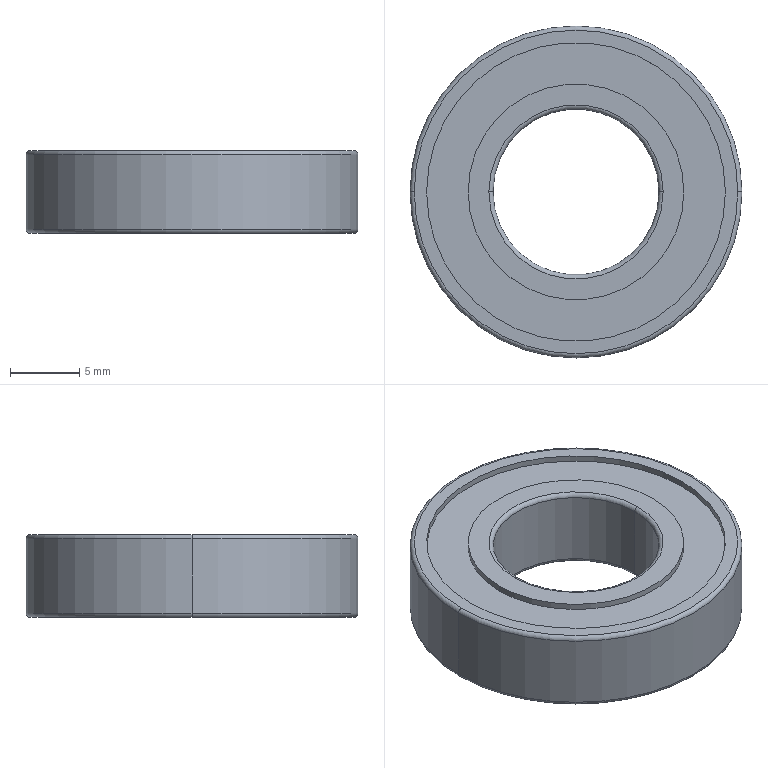Component | SolidWorks | TensioningWheel-2-1_B6901ZZ-2-2 | 1 solid | 26 faces | box 24 x 24 x 6 mm | volume 1874 mm3 | cylinder 12 | torus 8 | plane 6 | commonest cylinder face diameters 21.6 x4 15.6 x4 24 x2 12 x2
build123d program:
from build123d import *


with BuildPart() as part:
    # Sketch1 → Revolve1 (revolve)
    with BuildSketch(Plane.XY, mode=Mode.PRIVATE) as revolve1_sk:
        with BuildLine():
            Line((0, 11.7), (0, 10.8))
            Line((0, 10.8), (0.45, 10.8))
            Line((0.45, 10.8), (0.45, 7.8))
            Line((0.45, 7.8), (0, 7.8))
            Line((0, 7.8), (0, 6.3))
            ThreePointArc((0, 6.3), (0.08787, 6.088), (0.3, 6))
            Line((0.3, 6), (5.7, 6))
            ThreePointArc((5.7, 6), (5.912, 6.088), (6, 6.3))
            Line((6, 6.3), (6, 7.8))
            Line((6, 7.8), (5.55, 7.8))
            Line((5.55, 7.8), (5.55, 10.8))
            Line((5.55, 10.8), (6, 10.8))
            Line((6, 10.8), (6, 11.7))
            ThreePointArc((6, 11.7), (5.912, 11.912), (5.7, 12))
            Line((5.7, 12), (0.3, 12))
            ThreePointArc((0.3, 12), (0.08787, 11.912), (0, 11.7))
        make_face()
    revolve(revolve1_sk.sketch.rotate(Axis((6, 0, 0), (-1, 0, 0)), 270), axis=Axis((6, 0, 0), (-1, 0, 0)))


solid = part.part

# Placed as in the assembly
solid = solid.moved(Location((538.036, -118.615, -116), (0, 90, 0)))
STEP:
#1=COLOUR_RGB('',0.7922,0.8196,0.9333);
#2=FILL_AREA_STYLE_COLOUR('',#1);
#3=FILL_AREA_STYLE('',(#2));
#4=SURFACE_STYLE_FILL_AREA(#3);
#5=SURFACE_SIDE_STYLE('',(#4));
#6=SURFACE_STYLE_USAGE(.BOTH.,#5);
#7=PRESENTATION_STYLE_ASSIGNMENT((#6));
#8=CARTESIAN_POINT('',(20.71,-4.67,-4.579));
#9=VERTEX_POINT('',#8);
#10=CARTESIAN_POINT('',(21.655,-4.67,-4.579));
#11=VERTEX_POINT('',#10);
#12=CARTESIAN_POINT('',(21.183,-4.67,-4.579));
#13=DIRECTION('',(0.,0.,-1.));
#14=DIRECTION('',(-1.,0.,0.));
#15=AXIS2_PLACEMENT_3D('',#12,#13,#14);
#16=CIRCLE('',#15,0.4724);
#17=EDGE_CURVE('',#9,#11,#16,.T.);
#18=ORIENTED_EDGE('',*,*,#17,.T.);
#19=CARTESIAN_POINT('',(21.655,-4.67,-4.791));
#20=VERTEX_POINT('',#19);
#21=CARTESIAN_POINT('',(21.655,-4.67,-4.567));
#22=DIRECTION('',(0.,0.,-1.));
#23=VECTOR('',#22,39.37);
#24=LINE('',#21,#23);
#25=EDGE_CURVE('',#11,#20,#24,.T.);
#26=ORIENTED_EDGE('',*,*,#25,.T.);
#27=CARTESIAN_POINT('',(20.71,-4.67,-4.791));
#28=VERTEX_POINT('',#27);
#29=CARTESIAN_POINT('',(21.183,-4.67,-4.791));
#30=DIRECTION('',(0.,0.,-1.));
#31=DIRECTION('',(-1.,0.,0.));
#32=AXIS2_PLACEMENT_3D('',#29,#30,#31);
#33=CIRCLE('',#32,0.4724);
#34=EDGE_CURVE('',#28,#20,#33,.T.);
#35=ORIENTED_EDGE('',*,*,#34,.F.);
#36=CARTESIAN_POINT('',(20.71,-4.67,-4.567));
#37=DIRECTION('',(0.,0.,-1.));
#38=VECTOR('',#37,39.37);
#39=LINE('',#36,#38);
#40=EDGE_CURVE('',#9,#28,#39,.T.);
#41=ORIENTED_EDGE('',*,*,#40,.F.);
#42=EDGE_LOOP('',(#18,#26,#35,#41));
#43=FACE_OUTER_BOUND('',#42,.T.);
#44=CARTESIAN_POINT('',(21.183,-4.67,-4.567));
#45=DIRECTION('',(0.,0.,-1.));
#46=DIRECTION('',(-1.,0.,0.));
#47=AXIS2_PLACEMENT_3D('',#44,#45,#46);
#48=CYLINDRICAL_SURFACE('',#47,0.4724);
#49=ADVANCED_FACE('',(#43),#48,.T.);
#50=CARTESIAN_POINT('',(20.722,-4.67,-4.567));
#51=VERTEX_POINT('',#50);
#52=CARTESIAN_POINT('',(21.643,-4.67,-4.567));
#53=VERTEX_POINT('',#52);
#54=CARTESIAN_POINT('',(21.183,-4.67,-4.567));
#55=DIRECTION('',(0.,0.,-1.));
#56=DIRECTION('',(-1.,0.,0.));
#57=AXIS2_PLACEMENT_3D('',#54,#55,#56);
#58=CIRCLE('',#57,0.4606);
#59=EDGE_CURVE('',#51,#53,#58,.T.);
#60=ORIENTED_EDGE('',*,*,#59,.T.);
#61=CARTESIAN_POINT('',(21.643,-4.67,-4.579));
#62=DIRECTION('',(-0.,1.,0.));
#63=DIRECTION('',(-1.,0.,0.));
#64=AXIS2_PLACEMENT_3D('',#61,#62,#63);
#65=CIRCLE('',#64,0.01181);
#66=EDGE_CURVE('',#53,#11,#65,.T.);
#67=ORIENTED_EDGE('',*,*,#66,.T.);
#68=ORIENTED_EDGE('',*,*,#17,.F.);
#69=CARTESIAN_POINT('',(20.722,-4.67,-4.579));
#70=DIRECTION('',(-0.,-1.,-0.));
#71=DIRECTION('',(0.,0.,-1.));
#72=AXIS2_PLACEMENT_3D('',#69,#70,#71);
#73=CIRCLE('',#72,0.01181);
#74=EDGE_CURVE('',#51,#9,#73,.T.);
#75=ORIENTED_EDGE('',*,*,#74,.F.);
#76=EDGE_LOOP('',(#60,#67,#68,#75));
#77=FACE_OUTER_BOUND('',#76,.T.);
#78=CARTESIAN_POINT('',(21.183,-4.67,-4.579));
#79=DIRECTION('',(0.,0.,-1.));
#80=DIRECTION('',(-1.,0.,-0.));
#81=AXIS2_PLACEMENT_3D('',#78,#79,#80);
#82=TOROIDAL_SURFACE('',#81,0.4606,0.01181);
#83=ADVANCED_FACE('',(#77),#82,.T.);
#84=CARTESIAN_POINT('',(21.608,-4.67,-4.567));
#85=VERTEX_POINT('',#84);
#86=CARTESIAN_POINT('',(20.757,-4.67,-4.567));
#87=VERTEX_POINT('',#86);
#88=CARTESIAN_POINT('',(21.183,-4.67,-4.567));
#89=DIRECTION('',(0.,0.,-1.));
#90=DIRECTION('',(-1.,0.,0.));
#91=AXIS2_PLACEMENT_3D('',#88,#89,#90);
#92=CIRCLE('',#91,0.4252);
#93=EDGE_CURVE('',#85,#87,#92,.T.);
#94=ORIENTED_EDGE('',*,*,#93,.F.);
#95=CARTESIAN_POINT('',(21.608,-4.67,-4.585));
#96=VERTEX_POINT('',#95);
#97=CARTESIAN_POINT('',(21.608,-4.67,-4.567));
#98=DIRECTION('',(0.,0.,-1.));
#99=VECTOR('',#98,39.37);
#100=LINE('',#97,#99);
#101=EDGE_CURVE('',#85,#96,#100,.T.);
#102=ORIENTED_EDGE('',*,*,#101,.T.);
#103=CARTESIAN_POINT('',(20.757,-4.67,-4.585));
#104=VERTEX_POINT('',#103);
#105=CARTESIAN_POINT('',(21.183,-4.67,-4.585));
#106=DIRECTION('',(0.,0.,-1.));
#107=DIRECTION('',(-1.,0.,0.));
#108=AXIS2_PLACEMENT_3D('',#105,#106,#107);
#109=CIRCLE('',#108,0.4252);
#110=EDGE_CURVE('',#96,#104,#109,.T.);
#111=ORIENTED_EDGE('',*,*,#110,.T.);
#112=CARTESIAN_POINT('',(20.757,-4.67,-4.567));
#113=DIRECTION('',(0.,0.,-1.));
#114=VECTOR('',#113,39.37);
#115=LINE('',#112,#114);
#116=EDGE_CURVE('',#87,#104,#115,.T.);
#117=ORIENTED_EDGE('',*,*,#116,.F.);
#118=EDGE_LOOP('',(#94,#102,#111,#117));
#119=FACE_OUTER_BOUND('',#118,.T.);
#120=CARTESIAN_POINT('',(21.183,-4.67,-4.567));
#121=DIRECTION('',(0.,0.,-1.));
#122=DIRECTION('',(-1.,0.,0.));
#123=AXIS2_PLACEMENT_3D('',#120,#121,#122);
#124=CYLINDRICAL_SURFACE('',#123,0.4252);
#125=ADVANCED_FACE('',(#119),#124,.F.);
#126=CARTESIAN_POINT('',(20.875,-4.67,-4.567));
#127=VERTEX_POINT('',#126);
#128=CARTESIAN_POINT('',(21.49,-4.67,-4.567));
#129=VERTEX_POINT('',#128);
#130=CARTESIAN_POINT('',(21.183,-4.67,-4.567));
#131=DIRECTION('',(0.,0.,-1.));
#132=DIRECTION('',(-1.,0.,0.));
#133=AXIS2_PLACEMENT_3D('',#130,#131,#132);
#134=CIRCLE('',#133,0.3071);
#135=EDGE_CURVE('',#127,#129,#134,.T.);
#136=ORIENTED_EDGE('',*,*,#135,.T.);
#137=CARTESIAN_POINT('',(21.49,-4.67,-4.585));
#138=VERTEX_POINT('',#137);
#139=CARTESIAN_POINT('',(21.49,-4.67,-4.567));
#140=DIRECTION('',(0.,0.,-1.));
#141=VECTOR('',#140,39.37);
#142=LINE('',#139,#141);
#143=EDGE_CURVE('',#129,#138,#142,.T.);
#144=ORIENTED_EDGE('',*,*,#143,.T.);
#145=CARTESIAN_POINT('',(20.875,-4.67,-4.585));
#146=VERTEX_POINT('',#145);
#147=CARTESIAN_POINT('',(21.183,-4.67,-4.585));
#148=DIRECTION('',(0.,0.,-1.));
#149=DIRECTION('',(-1.,0.,0.));
#150=AXIS2_PLACEMENT_3D('',#147,#148,#149);
#151=CIRCLE('',#150,0.3071);
#152=EDGE_CURVE('',#146,#138,#151,.T.);
#153=ORIENTED_EDGE('',*,*,#152,.F.);
#154=CARTESIAN_POINT('',(20.875,-4.67,-4.567));
#155=DIRECTION('',(0.,0.,-1.));
#156=VECTOR('',#155,39.37);
#157=LINE('',#154,#156);
#158=EDGE_CURVE('',#127,#146,#157,.T.);
#159=ORIENTED_EDGE('',*,*,#158,.F.);
#160=EDGE_LOOP('',(#136,#144,#153,#159));
#161=FACE_OUTER_BOUND('',#160,.T.);
#162=CARTESIAN_POINT('',(21.183,-4.67,-4.567));
#163=DIRECTION('',(0.,0.,-1.));
#164=DIRECTION('',(-1.,0.,0.));
#165=AXIS2_PLACEMENT_3D('',#162,#163,#164);
#166=CYLINDRICAL_SURFACE('',#165,0.3071);
#167=ADVANCED_FACE('',(#161),#166,.T.);
#168=CARTESIAN_POINT('',(20.946,-4.67,-4.579));
#169=VERTEX_POINT('',#168);
#170=CARTESIAN_POINT('',(21.419,-4.67,-4.579));
#171=VERTEX_POINT('',#170);
#172=CARTESIAN_POINT('',(21.183,-4.67,-4.579));
#173=DIRECTION('',(0.,0.,-1.));
#174=DIRECTION('',(-1.,0.,0.));
#175=AXIS2_PLACEMENT_3D('',#172,#173,#174);
#176=CIRCLE('',#175,0.2362);
#177=EDGE_CURVE('',#169,#171,#176,.T.);
#178=ORIENTED_EDGE('',*,*,#177,.T.);
#179=CARTESIAN_POINT('',(21.431,-4.67,-4.567));
#180=VERTEX_POINT('',#179);
#181=CARTESIAN_POINT('',(21.431,-4.67,-4.579));
#182=DIRECTION('',(-0.,1.,0.));
#183=DIRECTION('',(-1.,0.,0.));
#184=AXIS2_PLACEMENT_3D('',#181,#182,#183);
#185=CIRCLE('',#184,0.01181);
#186=EDGE_CURVE('',#171,#180,#185,.T.);
#187=ORIENTED_EDGE('',*,*,#186,.T.);
#188=CARTESIAN_POINT('',(20.934,-4.67,-4.567));
#189=VERTEX_POINT('',#188);
#190=CARTESIAN_POINT('',(21.183,-4.67,-4.567));
#191=DIRECTION('',(0.,0.,-1.));
#192=DIRECTION('',(-1.,0.,0.));
#193=AXIS2_PLACEMENT_3D('',#190,#191,#192);
#194=CIRCLE('',#193,0.248);
#195=EDGE_CURVE('',#189,#180,#194,.T.);
#196=ORIENTED_EDGE('',*,*,#195,.F.);
#197=CARTESIAN_POINT('',(20.934,-4.67,-4.579));
#198=DIRECTION('',(-0.,-1.,-0.));
#199=DIRECTION('',(0.,0.,-1.));
#200=AXIS2_PLACEMENT_3D('',#197,#198,#199);
#201=CIRCLE('',#200,0.01181);
#202=EDGE_CURVE('',#169,#189,#201,.T.);
#203=ORIENTED_EDGE('',*,*,#202,.F.);
#204=EDGE_LOOP('',(#178,#187,#196,#203));
#205=FACE_OUTER_BOUND('',#204,.T.);
#206=CARTESIAN_POINT('',(21.183,-4.67,-4.579));
#207=DIRECTION('',(0.,0.,-1.));
#208=DIRECTION('',(-1.,0.,-0.));
#209=AXIS2_PLACEMENT_3D('',#206,#207,#208);
#210=TOROIDAL_SURFACE('',#209,0.248,0.01181);
#211=ADVANCED_FACE('',(#205),#210,.T.);
#212=CARTESIAN_POINT('',(21.183,-4.67,-4.579));
#213=DIRECTION('',(0.,0.,-1.));
#214=DIRECTION('',(-1.,0.,0.));
#215=AXIS2_PLACEMENT_3D('',#212,#213,#214);
#216=CIRCLE('',#215,0.2362);
#217=EDGE_CURVE('',#171,#169,#216,.T.);
#218=ORIENTED_EDGE('',*,*,#217,.F.);
#219=CARTESIAN_POINT('',(21.419,-4.67,-4.791));
#220=VERTEX_POINT('',#219);
#221=CARTESIAN_POINT('',(21.419,-4.67,-4.567));
#222=DIRECTION('',(0.,0.,-1.));
#223=VECTOR('',#222,39.37);
#224=LINE('',#221,#223);
#225=EDGE_CURVE('',#171,#220,#224,.T.);
#226=ORIENTED_EDGE('',*,*,#225,.T.);
#227=CARTESIAN_POINT('',(20.946,-4.67,-4.791));
#228=VERTEX_POINT('',#227);
#229=CARTESIAN_POINT('',(21.183,-4.67,-4.791));
#230=DIRECTION('',(0.,0.,-1.));
#231=DIRECTION('',(-1.,0.,0.));
#232=AXIS2_PLACEMENT_3D('',#229,#230,#231);
#233=CIRCLE('',#232,0.2362);
#234=EDGE_CURVE('',#220,#228,#233,.T.);
#235=ORIENTED_EDGE('',*,*,#234,.T.);
#236=CARTESIAN_POINT('',(20.946,-4.67,-4.567));
#237=DIRECTION('',(0.,0.,-1.));
#238=VECTOR('',#237,39.37);
#239=LINE('',#236,#238);
#240=EDGE_CURVE('',#169,#228,#239,.T.);
#241=ORIENTED_EDGE('',*,*,#240,.F.);
#242=EDGE_LOOP('',(#218,#226,#235,#241));
#243=FACE_OUTER_BOUND('',#242,.T.);
#244=CARTESIAN_POINT('',(21.183,-4.67,-4.567));
#245=DIRECTION('',(0.,0.,-1.));
#246=DIRECTION('',(-1.,0.,0.));
#247=AXIS2_PLACEMENT_3D('',#244,#245,#246);
#248=CYLINDRICAL_SURFACE('',#247,0.2362);
#249=ADVANCED_FACE('',(#243),#248,.F.);
#250=CARTESIAN_POINT('',(20.934,-4.67,-4.803));
#251=VERTEX_POINT('',#250);
#252=CARTESIAN_POINT('',(21.431,-4.67,-4.803));
#253=VERTEX_POINT('',#252);
#254=CARTESIAN_POINT('',(21.183,-4.67,-4.803));
#255=DIRECTION('',(0.,0.,-1.));
#256=DIRECTION('',(-1.,0.,0.));
#257=AXIS2_PLACEMENT_3D('',#254,#255,#256);
#258=CIRCLE('',#257,0.248);
#259=EDGE_CURVE('',#251,#253,#258,.T.);
#260=ORIENTED_EDGE('',*,*,#259,.T.);
#261=CARTESIAN_POINT('',(21.431,-4.67,-4.791));
#262=DIRECTION('',(-0.,1.,0.));
#263=DIRECTION('',(-1.,0.,0.));
#264=AXIS2_PLACEMENT_3D('',#261,#262,#263);
#265=CIRCLE('',#264,0.01181);
#266=EDGE_CURVE('',#253,#220,#265,.T.);
#267=ORIENTED_EDGE('',*,*,#266,.T.);
#268=CARTESIAN_POINT('',(21.183,-4.67,-4.791));
#269=DIRECTION('',(0.,0.,-1.));
#270=DIRECTION('',(-1.,0.,0.));
#271=AXIS2_PLACEMENT_3D('',#268,#269,#270);
#272=CIRCLE('',#271,0.2362);
#273=EDGE_CURVE('',#228,#220,#272,.T.);
#274=ORIENTED_EDGE('',*,*,#273,.F.);
#275=CARTESIAN_POINT('',(20.934,-4.67,-4.791));
#276=DIRECTION('',(-0.,-1.,-0.));
#277=DIRECTION('',(0.,0.,-1.));
#278=AXIS2_PLACEMENT_3D('',#275,#276,#277);
#279=CIRCLE('',#278,0.01181);
#280=EDGE_CURVE('',#251,#228,#279,.T.);
#281=ORIENTED_EDGE('',*,*,#280,.F.);
#282=EDGE_LOOP('',(#260,#267,#274,#281));
#283=FACE_OUTER_BOUND('',#282,.T.);
#284=CARTESIAN_POINT('',(21.183,-4.67,-4.791));
#285=DIRECTION('',(0.,0.,-1.));
#286=DIRECTION('',(-1.,0.,-0.));
#287=AXIS2_PLACEMENT_3D('',#284,#285,#286);
#288=TOROIDAL_SURFACE('',#287,0.248,0.01181);
#289=ADVANCED_FACE('',(#283),#288,.T.);
#290=CARTESIAN_POINT('',(20.875,-4.67,-4.785));
#291=VERTEX_POINT('',#290);
#292=CARTESIAN_POINT('',(21.49,-4.67,-4.785));
#293=VERTEX_POINT('',#292);
#294=CARTESIAN_POINT('',(21.183,-4.67,-4.785));
#295=DIRECTION('',(0.,0.,-1.));
#296=DIRECTION('',(-1.,0.,0.));
#297=AXIS2_PLACEMENT_3D('',#294,#295,#296);
#298=CIRCLE('',#297,0.3071);
#299=EDGE_CURVE('',#291,#293,#298,.T.);
#300=ORIENTED_EDGE('',*,*,#299,.T.);
#301=CARTESIAN_POINT('',(21.49,-4.67,-4.803));
#302=VERTEX_POINT('',#301);
#303=CARTESIAN_POINT('',(21.49,-4.67,-4.567));
#304=DIRECTION('',(0.,0.,-1.));
#305=VECTOR('',#304,39.37);
#306=LINE('',#303,#305);
#307=EDGE_CURVE('',#293,#302,#306,.T.);
#308=ORIENTED_EDGE('',*,*,#307,.T.);
#309=CARTESIAN_POINT('',(20.875,-4.67,-4.803));
#310=VERTEX_POINT('',#309);
#311=CARTESIAN_POINT('',(21.183,-4.67,-4.803));
#312=DIRECTION('',(0.,0.,-1.));
#313=DIRECTION('',(-1.,0.,0.));
#314=AXIS2_PLACEMENT_3D('',#311,#312,#313);
#315=CIRCLE('',#314,0.3071);
#316=EDGE_CURVE('',#310,#302,#315,.T.);
#317=ORIENTED_EDGE('',*,*,#316,.F.);
#318=CARTESIAN_POINT('',(20.875,-4.67,-4.567));
#319=DIRECTION('',(0.,0.,-1.));
#320=VECTOR('',#319,39.37);
#321=LINE('',#318,#320);
#322=EDGE_CURVE('',#291,#310,#321,.T.);
#323=ORIENTED_EDGE('',*,*,#322,.F.);
#324=EDGE_LOOP('',(#300,#308,#317,#323));
#325=FACE_OUTER_BOUND('',#324,.T.);
#326=CARTESIAN_POINT('',(21.183,-4.67,-4.567));
#327=DIRECTION('',(0.,0.,-1.));
#328=DIRECTION('',(-1.,0.,0.));
#329=AXIS2_PLACEMENT_3D('',#326,#327,#328);
#330=CYLINDRICAL_SURFACE('',#329,0.3071);
#331=ADVANCED_FACE('',(#325),#330,.T.);
#332=CARTESIAN_POINT('',(21.608,-4.67,-4.785));
#333=VERTEX_POINT('',#332);
#334=CARTESIAN_POINT('',(20.757,-4.67,-4.785));
#335=VERTEX_POINT('',#334);
#336=CARTESIAN_POINT('',(21.183,-4.67,-4.785));
#337=DIRECTION('',(0.,0.,-1.));
#338=DIRECTION('',(-1.,0.,0.));
#339=AXIS2_PLACEMENT_3D('',#336,#337,#338);
#340=CIRCLE('',#339,0.4252);
#341=EDGE_CURVE('',#333,#335,#340,.T.);
#342=ORIENTED_EDGE('',*,*,#341,.F.);
#343=CARTESIAN_POINT('',(21.608,-4.67,-4.803));
#344=VERTEX_POINT('',#343);
#345=CARTESIAN_POINT('',(21.608,-4.67,-4.567));
#346=DIRECTION('',(0.,0.,-1.));
#347=VECTOR('',#346,39.37);
#348=LINE('',#345,#347);
#349=EDGE_CURVE('',#333,#344,#348,.T.);
#350=ORIENTED_EDGE('',*,*,#349,.T.);
#351=CARTESIAN_POINT('',(20.757,-4.67,-4.803));
#352=VERTEX_POINT('',#351);
#353=CARTESIAN_POINT('',(21.183,-4.67,-4.803));
#354=DIRECTION('',(0.,0.,-1.));
#355=DIRECTION('',(-1.,0.,0.));
#356=AXIS2_PLACEMENT_3D('',#353,#354,#355);
#357=CIRCLE('',#356,0.4252);
#358=EDGE_CURVE('',#344,#352,#357,.T.);
#359=ORIENTED_EDGE('',*,*,#358,.T.);
#360=CARTESIAN_POINT('',(20.757,-4.67,-4.567));
#361=DIRECTION('',(0.,0.,-1.));
#362=VECTOR('',#361,39.37);
#363=LINE('',#360,#362);
#364=EDGE_CURVE('',#335,#352,#363,.T.);
#365=ORIENTED_EDGE('',*,*,#364,.F.);
#366=EDGE_LOOP('',(#342,#350,#359,#365));
#367=FACE_OUTER_BOUND('',#366,.T.);
#368=CARTESIAN_POINT('',(21.183,-4.67,-4.567));
#369=DIRECTION('',(0.,0.,-1.));
#370=DIRECTION('',(-1.,0.,0.));
#371=AXIS2_PLACEMENT_3D('',#368,#369,#370);
#372=CYLINDRICAL_SURFACE('',#371,0.4252);
#373=ADVANCED_FACE('',(#367),#372,.F.);
#374=ORIENTED_EDGE('',*,*,#34,.T.);
#375=CARTESIAN_POINT('',(21.643,-4.67,-4.803));
#376=VERTEX_POINT('',#375);
#377=CARTESIAN_POINT('',(21.643,-4.67,-4.791));
#378=DIRECTION('',(-0.,1.,0.));
#379=DIRECTION('',(-1.,0.,0.));
#380=AXIS2_PLACEMENT_3D('',#377,#378,#379);
#381=CIRCLE('',#380,0.01181);
#382=EDGE_CURVE('',#20,#376,#381,.T.);
#383=ORIENTED_EDGE('',*,*,#382,.T.);
#384=CARTESIAN_POINT('',(20.722,-4.67,-4.803));
#385=VERTEX_POINT('',#384);
#386=CARTESIAN_POINT('',(21.183,-4.67,-4.803));
#387=DIRECTION('',(0.,0.,-1.));
#388=DIRECTION('',(-1.,0.,0.));
#389=AXIS2_PLACEMENT_3D('',#386,#387,#388);
#390=CIRCLE('',#389,0.4606);
#391=EDGE_CURVE('',#385,#376,#390,.T.);
#392=ORIENTED_EDGE('',*,*,#391,.F.);
#393=CARTESIAN_POINT('',(20.722,-4.67,-4.791));
#394=DIRECTION('',(-0.,-1.,-0.));
#395=DIRECTION('',(0.,0.,-1.));
#396=AXIS2_PLACEMENT_3D('',#393,#394,#395);
#397=CIRCLE('',#396,0.01181);
#398=EDGE_CURVE('',#28,#385,#397,.T.);
#399=ORIENTED_EDGE('',*,*,#398,.F.);
#400=EDGE_LOOP('',(#374,#383,#392,#399));
#401=FACE_OUTER_BOUND('',#400,.T.);
#402=CARTESIAN_POINT('',(21.183,-4.67,-4.791));
#403=DIRECTION('',(0.,0.,-1.));
#404=DIRECTION('',(-1.,0.,-0.));
#405=AXIS2_PLACEMENT_3D('',#402,#403,#404);
#406=TOROIDAL_SURFACE('',#405,0.4606,0.01181);
#407=ADVANCED_FACE('',(#401),#406,.T.);
#408=ORIENTED_EDGE('',*,*,#382,.F.);
#409=CARTESIAN_POINT('',(21.183,-4.67,-4.791));
#410=DIRECTION('',(0.,0.,-1.));
#411=DIRECTION('',(-1.,0.,0.));
#412=AXIS2_PLACEMENT_3D('',#409,#410,#411);
#413=CIRCLE('',#412,0.4724);
#414=EDGE_CURVE('',#20,#28,#413,.T.);
#415=ORIENTED_EDGE('',*,*,#414,.T.);
#416=ORIENTED_EDGE('',*,*,#398,.T.);
#417=CARTESIAN_POINT('',(21.183,-4.67,-4.803));
#418=DIRECTION('',(0.,0.,-1.));
#419=DIRECTION('',(-1.,0.,0.));
#420=AXIS2_PLACEMENT_3D('',#417,#418,#419);
#421=CIRCLE('',#420,0.4606);
#422=EDGE_CURVE('',#376,#385,#421,.T.);
#423=ORIENTED_EDGE('',*,*,#422,.F.);
#424=EDGE_LOOP('',(#408,#415,#416,#423));
#425=FACE_OUTER_BOUND('',#424,.T.);
#426=CARTESIAN_POINT('',(21.183,-4.67,-4.791));
#427=DIRECTION('',(0.,0.,-1.));
#428=DIRECTION('',(-1.,0.,-0.));
#429=AXIS2_PLACEMENT_3D('',#426,#427,#428);
#430=TOROIDAL_SURFACE('',#429,0.4606,0.01181);
#431=ADVANCED_FACE('',(#425),#430,.T.);
#432=CARTESIAN_POINT('',(21.183,-4.67,-4.803));
#433=DIRECTION('',(0.,0.,-1.));
#434=DIRECTION('',(-1.,0.,0.));
#435=AXIS2_PLACEMENT_3D('',#432,#433,#434);
#436=CIRCLE('',#435,0.4252);
#437=EDGE_CURVE('',#352,#344,#436,.T.);
#438=ORIENTED_EDGE('',*,*,#437,.F.);
#439=ORIENTED_EDGE('',*,*,#358,.F.);
#440=EDGE_LOOP('',(#438,#439));
#441=FACE_BOUND('',#440,.T.);
#442=ORIENTED_EDGE('',*,*,#391,.T.);
#443=ORIENTED_EDGE('',*,*,#422,.T.);
#444=EDGE_LOOP('',(#442,#443));
#445=FACE_OUTER_BOUND('',#444,.T.);
#446=CARTESIAN_POINT('',(21.183,-4.209,-4.803));
#447=DIRECTION('',(-0.,-0.,1.));
#448=DIRECTION('',(1.,-0.,0.));
#449=AXIS2_PLACEMENT_3D('',#446,#447,#448);
#450=PLANE('',#449);
#451=ADVANCED_FACE('',(#441,#445),#450,.F.);
#452=ORIENTED_EDGE('',*,*,#349,.F.);
#453=CARTESIAN_POINT('',(21.183,-4.67,-4.785));
#454=DIRECTION('',(0.,0.,-1.));
#455=DIRECTION('',(-1.,0.,0.));
#456=AXIS2_PLACEMENT_3D('',#453,#454,#455);
#457=CIRCLE('',#456,0.4252);
#458=EDGE_CURVE('',#335,#333,#457,.T.);
#459=ORIENTED_EDGE('',*,*,#458,.F.);
#460=ORIENTED_EDGE('',*,*,#364,.T.);
#461=ORIENTED_EDGE('',*,*,#437,.T.);
#462=EDGE_LOOP('',(#452,#459,#460,#461));
#463=FACE_OUTER_BOUND('',#462,.T.);
#464=CARTESIAN_POINT('',(21.183,-4.67,-4.567));
#465=DIRECTION('',(0.,0.,-1.));
#466=DIRECTION('',(-1.,0.,0.));
#467=AXIS2_PLACEMENT_3D('',#464,#465,#466);
#468=CYLINDRICAL_SURFACE('',#467,0.4252);
#469=ADVANCED_FACE('',(#463),#468,.F.);
#470=ORIENTED_EDGE('',*,*,#299,.F.);
#471=CARTESIAN_POINT('',(21.183,-4.67,-4.785));
#472=DIRECTION('',(0.,0.,-1.));
#473=DIRECTION('',(-1.,0.,0.));
#474=AXIS2_PLACEMENT_3D('',#471,#472,#473);
#475=CIRCLE('',#474,0.3071);
#476=EDGE_CURVE('',#293,#291,#475,.T.);
#477=ORIENTED_EDGE('',*,*,#476,.F.);
#478=EDGE_LOOP('',(#470,#477));
#479=FACE_BOUND('',#478,.T.);
#480=ORIENTED_EDGE('',*,*,#458,.T.);
#481=ORIENTED_EDGE('',*,*,#341,.T.);
#482=EDGE_LOOP('',(#480,#481));
#483=FACE_OUTER_BOUND('',#482,.T.);
#484=CARTESIAN_POINT('',(21.183,-4.245,-4.785));
#485=DIRECTION('',(-0.,-0.,1.));
#486=DIRECTION('',(1.,-0.,0.));
#487=AXIS2_PLACEMENT_3D('',#484,#485,#486);
#488=PLANE('',#487);
#489=ADVANCED_FACE('',(#479,#483),#488,.F.);
#490=ORIENTED_EDGE('',*,*,#307,.F.);
#491=ORIENTED_EDGE('',*,*,#476,.T.);
#492=ORIENTED_EDGE('',*,*,#322,.T.);
#493=CARTESIAN_POINT('',(21.183,-4.67,-4.803));
#494=DIRECTION('',(0.,0.,-1.));
#495=DIRECTION('',(-1.,0.,0.));
#496=AXIS2_PLACEMENT_3D('',#493,#494,#495);
#497=CIRCLE('',#496,0.3071);
#498=EDGE_CURVE('',#302,#310,#497,.T.);
#499=ORIENTED_EDGE('',*,*,#498,.F.);
#500=EDGE_LOOP('',(#490,#491,#492,#499));
#501=FACE_OUTER_BOUND('',#500,.T.);
#502=CARTESIAN_POINT('',(21.183,-4.67,-4.567));
#503=DIRECTION('',(0.,0.,-1.));
#504=DIRECTION('',(-1.,0.,0.));
#505=AXIS2_PLACEMENT_3D('',#502,#503,#504);
#506=CYLINDRICAL_SURFACE('',#505,0.3071);
#507=ADVANCED_FACE('',(#501),#506,.T.);
#508=ORIENTED_EDGE('',*,*,#259,.F.);
#509=CARTESIAN_POINT('',(21.183,-4.67,-4.803));
#510=DIRECTION('',(0.,0.,-1.));
#511=DIRECTION('',(-1.,0.,0.));
#512=AXIS2_PLACEMENT_3D('',#509,#510,#511);
#513=CIRCLE('',#512,0.248);
#514=EDGE_CURVE('',#253,#251,#513,.T.);
#515=ORIENTED_EDGE('',*,*,#514,.F.);
#516=EDGE_LOOP('',(#508,#515));
#517=FACE_BOUND('',#516,.T.);
#518=ORIENTED_EDGE('',*,*,#316,.T.);
#519=ORIENTED_EDGE('',*,*,#498,.T.);
#520=EDGE_LOOP('',(#518,#519));
#521=FACE_OUTER_BOUND('',#520,.T.);
#522=CARTESIAN_POINT('',(21.183,-4.363,-4.803));
#523=DIRECTION('',(-0.,-0.,1.));
#524=DIRECTION('',(1.,-0.,0.));
#525=AXIS2_PLACEMENT_3D('',#522,#523,#524);
#526=PLANE('',#525);
#527=ADVANCED_FACE('',(#517,#521),#526,.F.);
#528=ORIENTED_EDGE('',*,*,#266,.F.);
#529=ORIENTED_EDGE('',*,*,#514,.T.);
#530=ORIENTED_EDGE('',*,*,#280,.T.);
#531=ORIENTED_EDGE('',*,*,#234,.F.);
#532=EDGE_LOOP('',(#528,#529,#530,#531));
#533=FACE_OUTER_BOUND('',#532,.T.);
#534=CARTESIAN_POINT('',(21.183,-4.67,-4.791));
#535=DIRECTION('',(0.,0.,-1.));
#536=DIRECTION('',(-1.,0.,-0.));
#537=AXIS2_PLACEMENT_3D('',#534,#535,#536);
#538=TOROIDAL_SURFACE('',#537,0.248,0.01181);
#539=ADVANCED_FACE('',(#533),#538,.T.);
#540=ORIENTED_EDGE('',*,*,#225,.F.);
#541=ORIENTED_EDGE('',*,*,#177,.F.);
#542=ORIENTED_EDGE('',*,*,#240,.T.);
#543=ORIENTED_EDGE('',*,*,#273,.T.);
#544=EDGE_LOOP('',(#540,#541,#542,#543));
#545=FACE_OUTER_BOUND('',#544,.T.);
#546=CARTESIAN_POINT('',(21.183,-4.67,-4.567));
#547=DIRECTION('',(0.,0.,-1.));
#548=DIRECTION('',(-1.,0.,0.));
#549=AXIS2_PLACEMENT_3D('',#546,#547,#548);
#550=CYLINDRICAL_SURFACE('',#549,0.2362);
#551=ADVANCED_FACE('',(#545),#550,.F.);
#552=ORIENTED_EDGE('',*,*,#186,.F.);
#553=ORIENTED_EDGE('',*,*,#217,.T.);
#554=ORIENTED_EDGE('',*,*,#202,.T.);
#555=CARTESIAN_POINT('',(21.183,-4.67,-4.567));
#556=DIRECTION('',(0.,0.,-1.));
#557=DIRECTION('',(-1.,0.,0.));
#558=AXIS2_PLACEMENT_3D('',#555,#556,#557);
#559=CIRCLE('',#558,0.248);
#560=EDGE_CURVE('',#180,#189,#559,.T.);
#561=ORIENTED_EDGE('',*,*,#560,.F.);
#562=EDGE_LOOP('',(#552,#553,#554,#561));
#563=FACE_OUTER_BOUND('',#562,.T.);
#564=CARTESIAN_POINT('',(21.183,-4.67,-4.579));
#565=DIRECTION('',(0.,0.,-1.));
#566=DIRECTION('',(-1.,0.,-0.));
#567=AXIS2_PLACEMENT_3D('',#564,#565,#566);
#568=TOROIDAL_SURFACE('',#567,0.248,0.01181);
#569=ADVANCED_FACE('',(#563),#568,.T.);
#570=ORIENTED_EDGE('',*,*,#135,.F.);
#571=CARTESIAN_POINT('',(21.183,-4.67,-4.567));
#572=DIRECTION('',(0.,0.,-1.));
#573=DIRECTION('',(-1.,0.,0.));
#574=AXIS2_PLACEMENT_3D('',#571,#572,#573);
#575=CIRCLE('',#574,0.3071);
#576=EDGE_CURVE('',#129,#127,#575,.T.);
#577=ORIENTED_EDGE('',*,*,#576,.F.);
#578=EDGE_LOOP('',(#570,#577));
#579=FACE_OUTER_BOUND('',#578,.T.);
#580=ORIENTED_EDGE('',*,*,#195,.T.);
#581=ORIENTED_EDGE('',*,*,#560,.T.);
#582=EDGE_LOOP('',(#580,#581));
#583=FACE_BOUND('',#582,.T.);
#584=CARTESIAN_POINT('',(21.183,-4.422,-4.567));
#585=DIRECTION('',(0.,0.,-1.));
#586=DIRECTION('',(-1.,0.,-0.));
#587=AXIS2_PLACEMENT_3D('',#584,#585,#586);
#588=PLANE('',#587);
#589=ADVANCED_FACE('',(#579,#583),#588,.F.);
#590=ORIENTED_EDGE('',*,*,#143,.F.);
#591=ORIENTED_EDGE('',*,*,#576,.T.);
#592=ORIENTED_EDGE('',*,*,#158,.T.);
#593=CARTESIAN_POINT('',(21.183,-4.67,-4.585));
#594=DIRECTION('',(0.,0.,-1.));
#595=DIRECTION('',(-1.,0.,0.));
#596=AXIS2_PLACEMENT_3D('',#593,#594,#595);
#597=CIRCLE('',#596,0.3071);
#598=EDGE_CURVE('',#138,#146,#597,.T.);
#599=ORIENTED_EDGE('',*,*,#598,.F.);
#600=EDGE_LOOP('',(#590,#591,#592,#599));
#601=FACE_OUTER_BOUND('',#600,.T.);
#602=CARTESIAN_POINT('',(21.183,-4.67,-4.567));
#603=DIRECTION('',(0.,0.,-1.));
#604=DIRECTION('',(-1.,0.,0.));
#605=AXIS2_PLACEMENT_3D('',#602,#603,#604);
#606=CYLINDRICAL_SURFACE('',#605,0.3071);
#607=ADVANCED_FACE('',(#601),#606,.T.);
#608=CARTESIAN_POINT('',(21.183,-4.67,-4.585));
#609=DIRECTION('',(0.,0.,-1.));
#610=DIRECTION('',(-1.,0.,0.));
#611=AXIS2_PLACEMENT_3D('',#608,#609,#610);
#612=CIRCLE('',#611,0.4252);
#613=EDGE_CURVE('',#104,#96,#612,.T.);
#614=ORIENTED_EDGE('',*,*,#613,.F.);
#615=ORIENTED_EDGE('',*,*,#110,.F.);
#616=EDGE_LOOP('',(#614,#615));
#617=FACE_OUTER_BOUND('',#616,.T.);
#618=ORIENTED_EDGE('',*,*,#152,.T.);
#619=ORIENTED_EDGE('',*,*,#598,.T.);
#620=EDGE_LOOP('',(#618,#619));
#621=FACE_BOUND('',#620,.T.);
#622=CARTESIAN_POINT('',(21.183,-4.363,-4.585));
#623=DIRECTION('',(0.,0.,-1.));
#624=DIRECTION('',(-1.,0.,-0.));
#625=AXIS2_PLACEMENT_3D('',#622,#623,#624);
#626=PLANE('',#625);
#627=ADVANCED_FACE('',(#617,#621),#626,.F.);
#628=ORIENTED_EDGE('',*,*,#101,.F.);
#629=CARTESIAN_POINT('',(21.183,-4.67,-4.567));
#630=DIRECTION('',(0.,0.,-1.));
#631=DIRECTION('',(-1.,0.,0.));
#632=AXIS2_PLACEMENT_3D('',#629,#630,#631);
#633=CIRCLE('',#632,0.4252);
#634=EDGE_CURVE('',#87,#85,#633,.T.);
#635=ORIENTED_EDGE('',*,*,#634,.F.);
#636=ORIENTED_EDGE('',*,*,#116,.T.);
#637=ORIENTED_EDGE('',*,*,#613,.T.);
#638=EDGE_LOOP('',(#628,#635,#636,#637));
#639=FACE_OUTER_BOUND('',#638,.T.);
#640=CARTESIAN_POINT('',(21.183,-4.67,-4.567));
#641=DIRECTION('',(0.,0.,-1.));
#642=DIRECTION('',(-1.,0.,0.));
#643=AXIS2_PLACEMENT_3D('',#640,#641,#642);
#644=CYLINDRICAL_SURFACE('',#643,0.4252);
#645=ADVANCED_FACE('',(#639),#644,.F.);
#646=ORIENTED_EDGE('',*,*,#59,.F.);
#647=CARTESIAN_POINT('',(21.183,-4.67,-4.567));
#648=DIRECTION('',(0.,0.,-1.));
#649=DIRECTION('',(-1.,0.,0.));
#650=AXIS2_PLACEMENT_3D('',#647,#648,#649);
#651=CIRCLE('',#650,0.4606);
#652=EDGE_CURVE('',#53,#51,#651,.T.);
#653=ORIENTED_EDGE('',*,*,#652,.F.);
#654=EDGE_LOOP('',(#646,#653));
#655=FACE_OUTER_BOUND('',#654,.T.);
#656=ORIENTED_EDGE('',*,*,#634,.T.);
#657=ORIENTED_EDGE('',*,*,#93,.T.);
#658=EDGE_LOOP('',(#656,#657));
#659=FACE_BOUND('',#658,.T.);
#660=CARTESIAN_POINT('',(21.183,-4.245,-4.567));
#661=DIRECTION('',(0.,0.,-1.));
#662=DIRECTION('',(-1.,0.,-0.));
#663=AXIS2_PLACEMENT_3D('',#660,#661,#662);
#664=PLANE('',#663);
#665=ADVANCED_FACE('',(#655,#659),#664,.F.);
#666=ORIENTED_EDGE('',*,*,#66,.F.);
#667=ORIENTED_EDGE('',*,*,#652,.T.);
#668=ORIENTED_EDGE('',*,*,#74,.T.);
#669=CARTESIAN_POINT('',(21.183,-4.67,-4.579));
#670=DIRECTION('',(0.,0.,-1.));
#671=DIRECTION('',(-1.,0.,0.));
#672=AXIS2_PLACEMENT_3D('',#669,#670,#671);
#673=CIRCLE('',#672,0.4724);
#674=EDGE_CURVE('',#11,#9,#673,.T.);
#675=ORIENTED_EDGE('',*,*,#674,.F.);
#676=EDGE_LOOP('',(#666,#667,#668,#675));
#677=FACE_OUTER_BOUND('',#676,.T.);
#678=CARTESIAN_POINT('',(21.183,-4.67,-4.579));
#679=DIRECTION('',(0.,0.,-1.));
#680=DIRECTION('',(-1.,0.,-0.));
#681=AXIS2_PLACEMENT_3D('',#678,#679,#680);
#682=TOROIDAL_SURFACE('',#681,0.4606,0.01181);
#683=ADVANCED_FACE('',(#677),#682,.T.);
#684=ORIENTED_EDGE('',*,*,#25,.F.);
#685=ORIENTED_EDGE('',*,*,#674,.T.);
#686=ORIENTED_EDGE('',*,*,#40,.T.);
#687=ORIENTED_EDGE('',*,*,#414,.F.);
#688=EDGE_LOOP('',(#684,#685,#686,#687));
#689=FACE_OUTER_BOUND('',#688,.T.);
#690=CARTESIAN_POINT('',(21.183,-4.67,-4.567));
#691=DIRECTION('',(0.,0.,-1.));
#692=DIRECTION('',(-1.,0.,0.));
#693=AXIS2_PLACEMENT_3D('',#690,#691,#692);
#694=CYLINDRICAL_SURFACE('',#693,0.4724);
#695=ADVANCED_FACE('',(#689),#694,.T.);
#696=CLOSED_SHELL('',(#49,#83,#125,#167,#211,#249,#289,#331,#373,#407,#431,#451,#469,#489,#507,#527,#539,#551,#569,#589,#607,#627,#645,#665,#683,#695));
#697=MANIFOLD_SOLID_BREP('',#696);
#698=STYLED_ITEM('',(#7),#697);
#699=PRESENTATION_LAYER_ASSIGNMENT('','',(#698));
#700=CARTESIAN_POINT('',(0.,0.,0.));
#701=DIRECTION('',(0.,0.,1.));
#702=DIRECTION('',(1.,0.,0.));
#703=AXIS2_PLACEMENT_3D('',#700,#701,#702);
#704=(LENGTH_UNIT()NAMED_UNIT(*)SI_UNIT($,.METRE.));
#705=LENGTH_MEASURE_WITH_UNIT(LENGTH_MEASURE(0.0254),#704);
#706=DIMENSIONAL_EXPONENTS(1.,0.,0.,0.,0.,0.,0.);
#707=(CONVERSION_BASED_UNIT('',#705)LENGTH_UNIT()NAMED_UNIT(#706));
#708=UNCERTAINTY_MEASURE_WITH_UNIT(LENGTH_MEASURE(0.00001),#707,'','');
#709=(NAMED_UNIT(*)PLANE_ANGLE_UNIT()SI_UNIT($,.RADIAN.));
#710=(NAMED_UNIT(*)SI_UNIT($,.STERADIAN.)SOLID_ANGLE_UNIT());
#711=(GEOMETRIC_REPRESENTATION_CONTEXT(3)GLOBAL_UNCERTAINTY_ASSIGNED_CONTEXT((#708))GLOBAL_UNIT_ASSIGNED_CONTEXT((#707,#709,#710))REPRESENTATION_CONTEXT('',''));
#712=ADVANCED_BREP_SHAPE_REPRESENTATION('',(#697,#703),#711);
#713=(LENGTH_UNIT()NAMED_UNIT(*)SI_UNIT($,.METRE.));
#714=LENGTH_MEASURE_WITH_UNIT(LENGTH_MEASURE(0.0254),#713);
#715=DIMENSIONAL_EXPONENTS(1.,0.,0.,0.,0.,0.,0.);
#716=(CONVERSION_BASED_UNIT('',#714)LENGTH_UNIT()NAMED_UNIT(#715));
#717=UNCERTAINTY_MEASURE_WITH_UNIT(LENGTH_MEASURE(0.00001),#716,'','');
#718=(NAMED_UNIT(*)PLANE_ANGLE_UNIT()SI_UNIT($,.RADIAN.));
#719=(NAMED_UNIT(*)SI_UNIT($,.STERADIAN.)SOLID_ANGLE_UNIT());
#720=(GEOMETRIC_REPRESENTATION_CONTEXT(3)GLOBAL_UNCERTAINTY_ASSIGNED_CONTEXT((#717))GLOBAL_UNIT_ASSIGNED_CONTEXT((#716,#718,#719))REPRESENTATION_CONTEXT('',''));
#721=MECHANICAL_DESIGN_GEOMETRIC_PRESENTATION_REPRESENTATION('',(#698),#720);